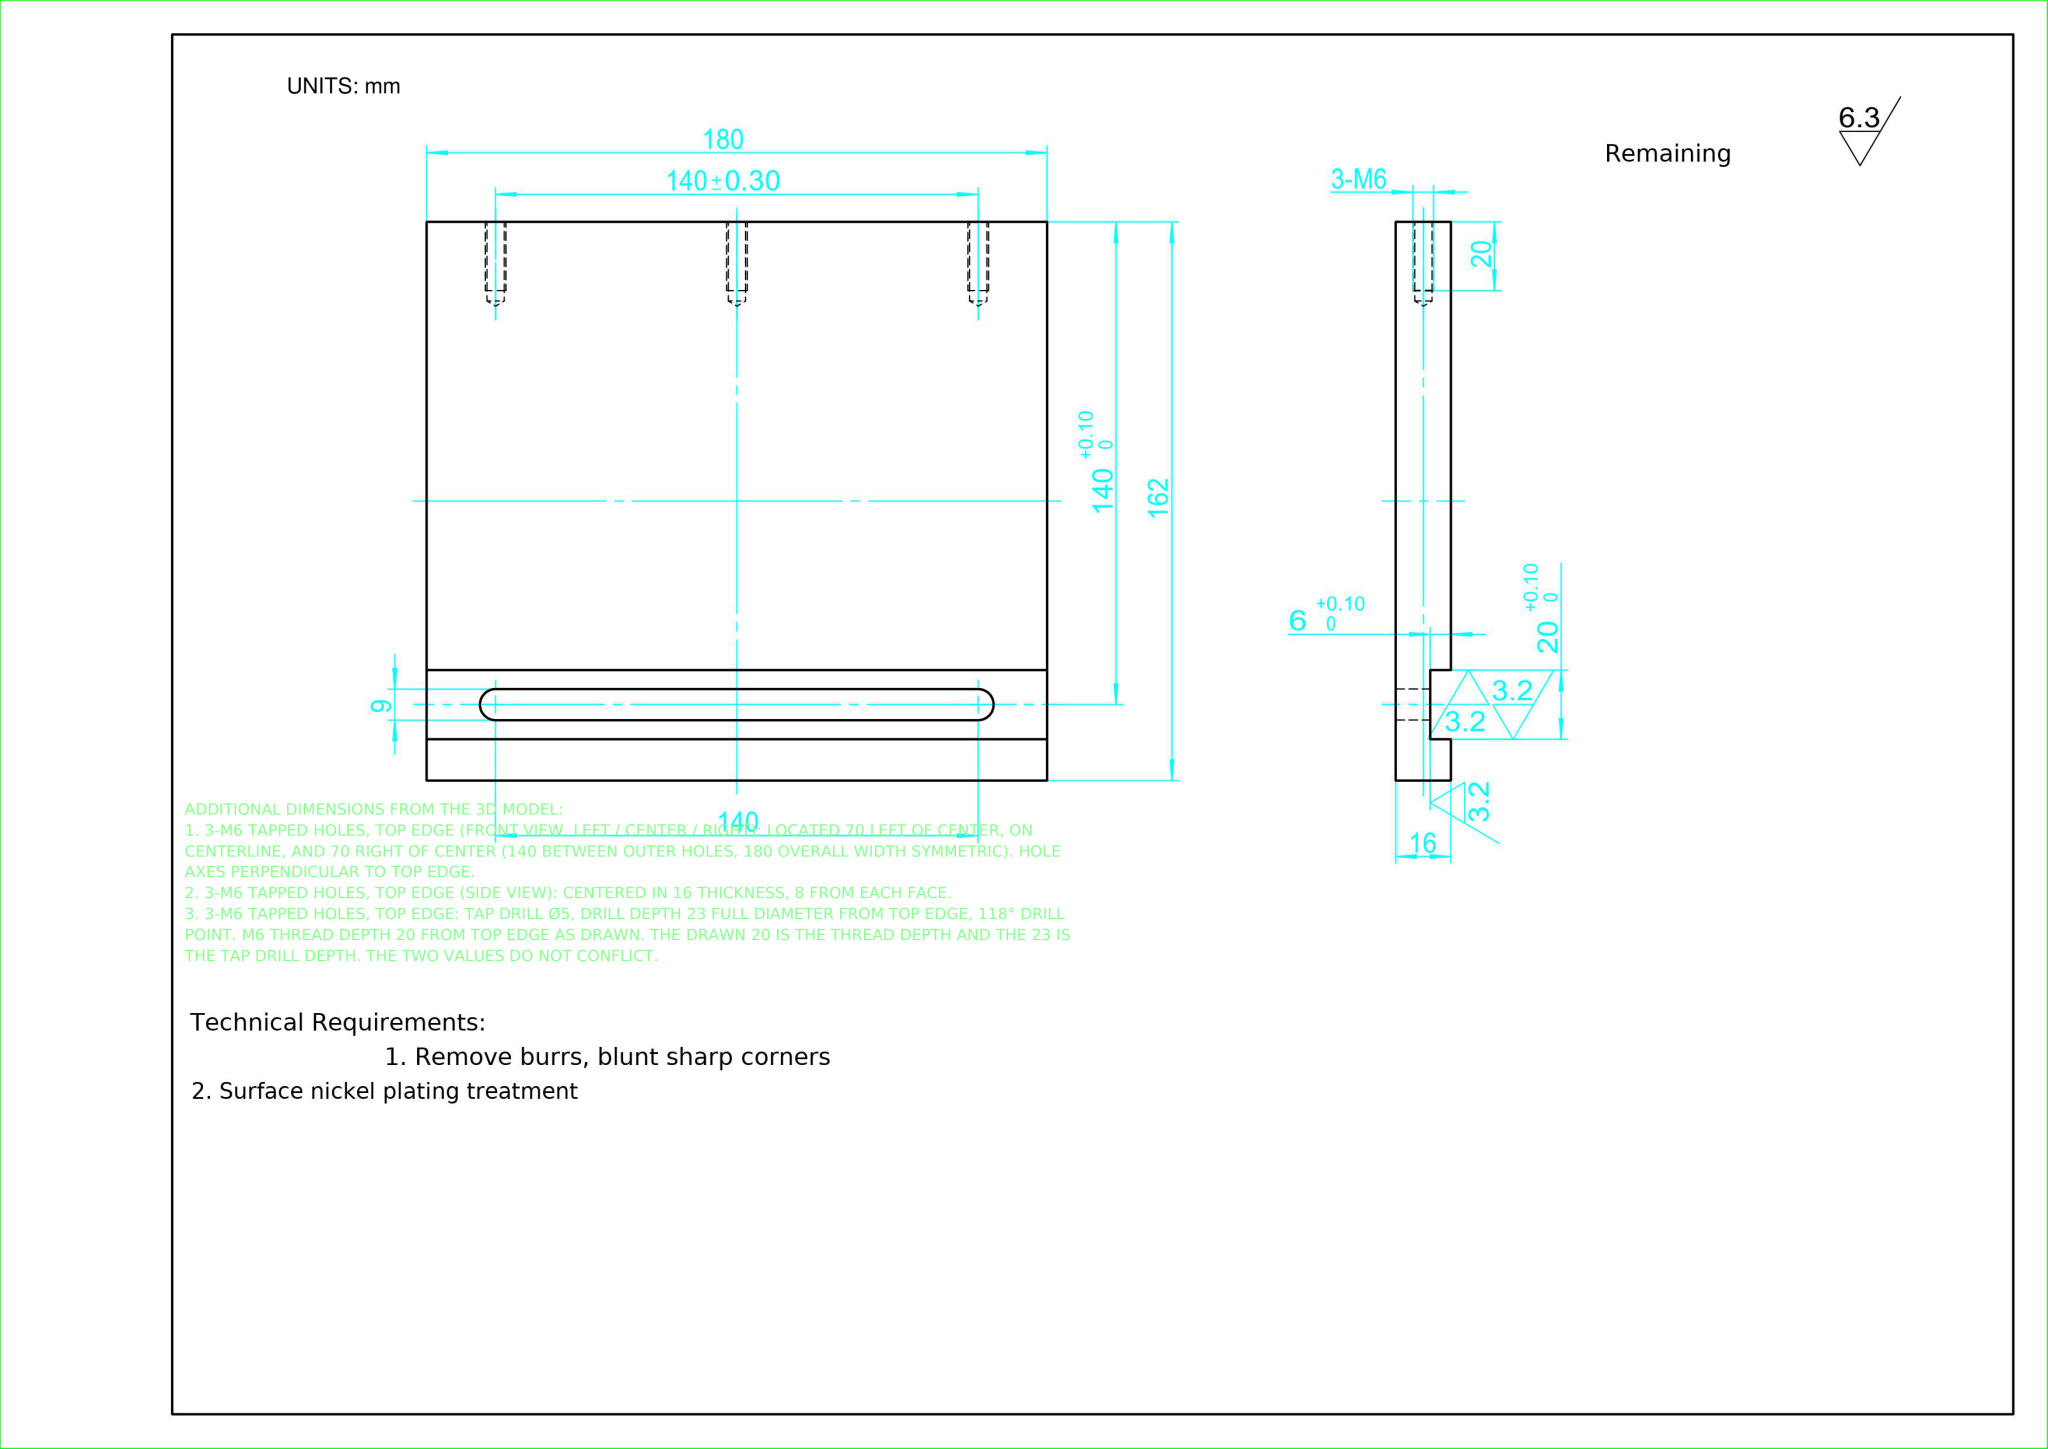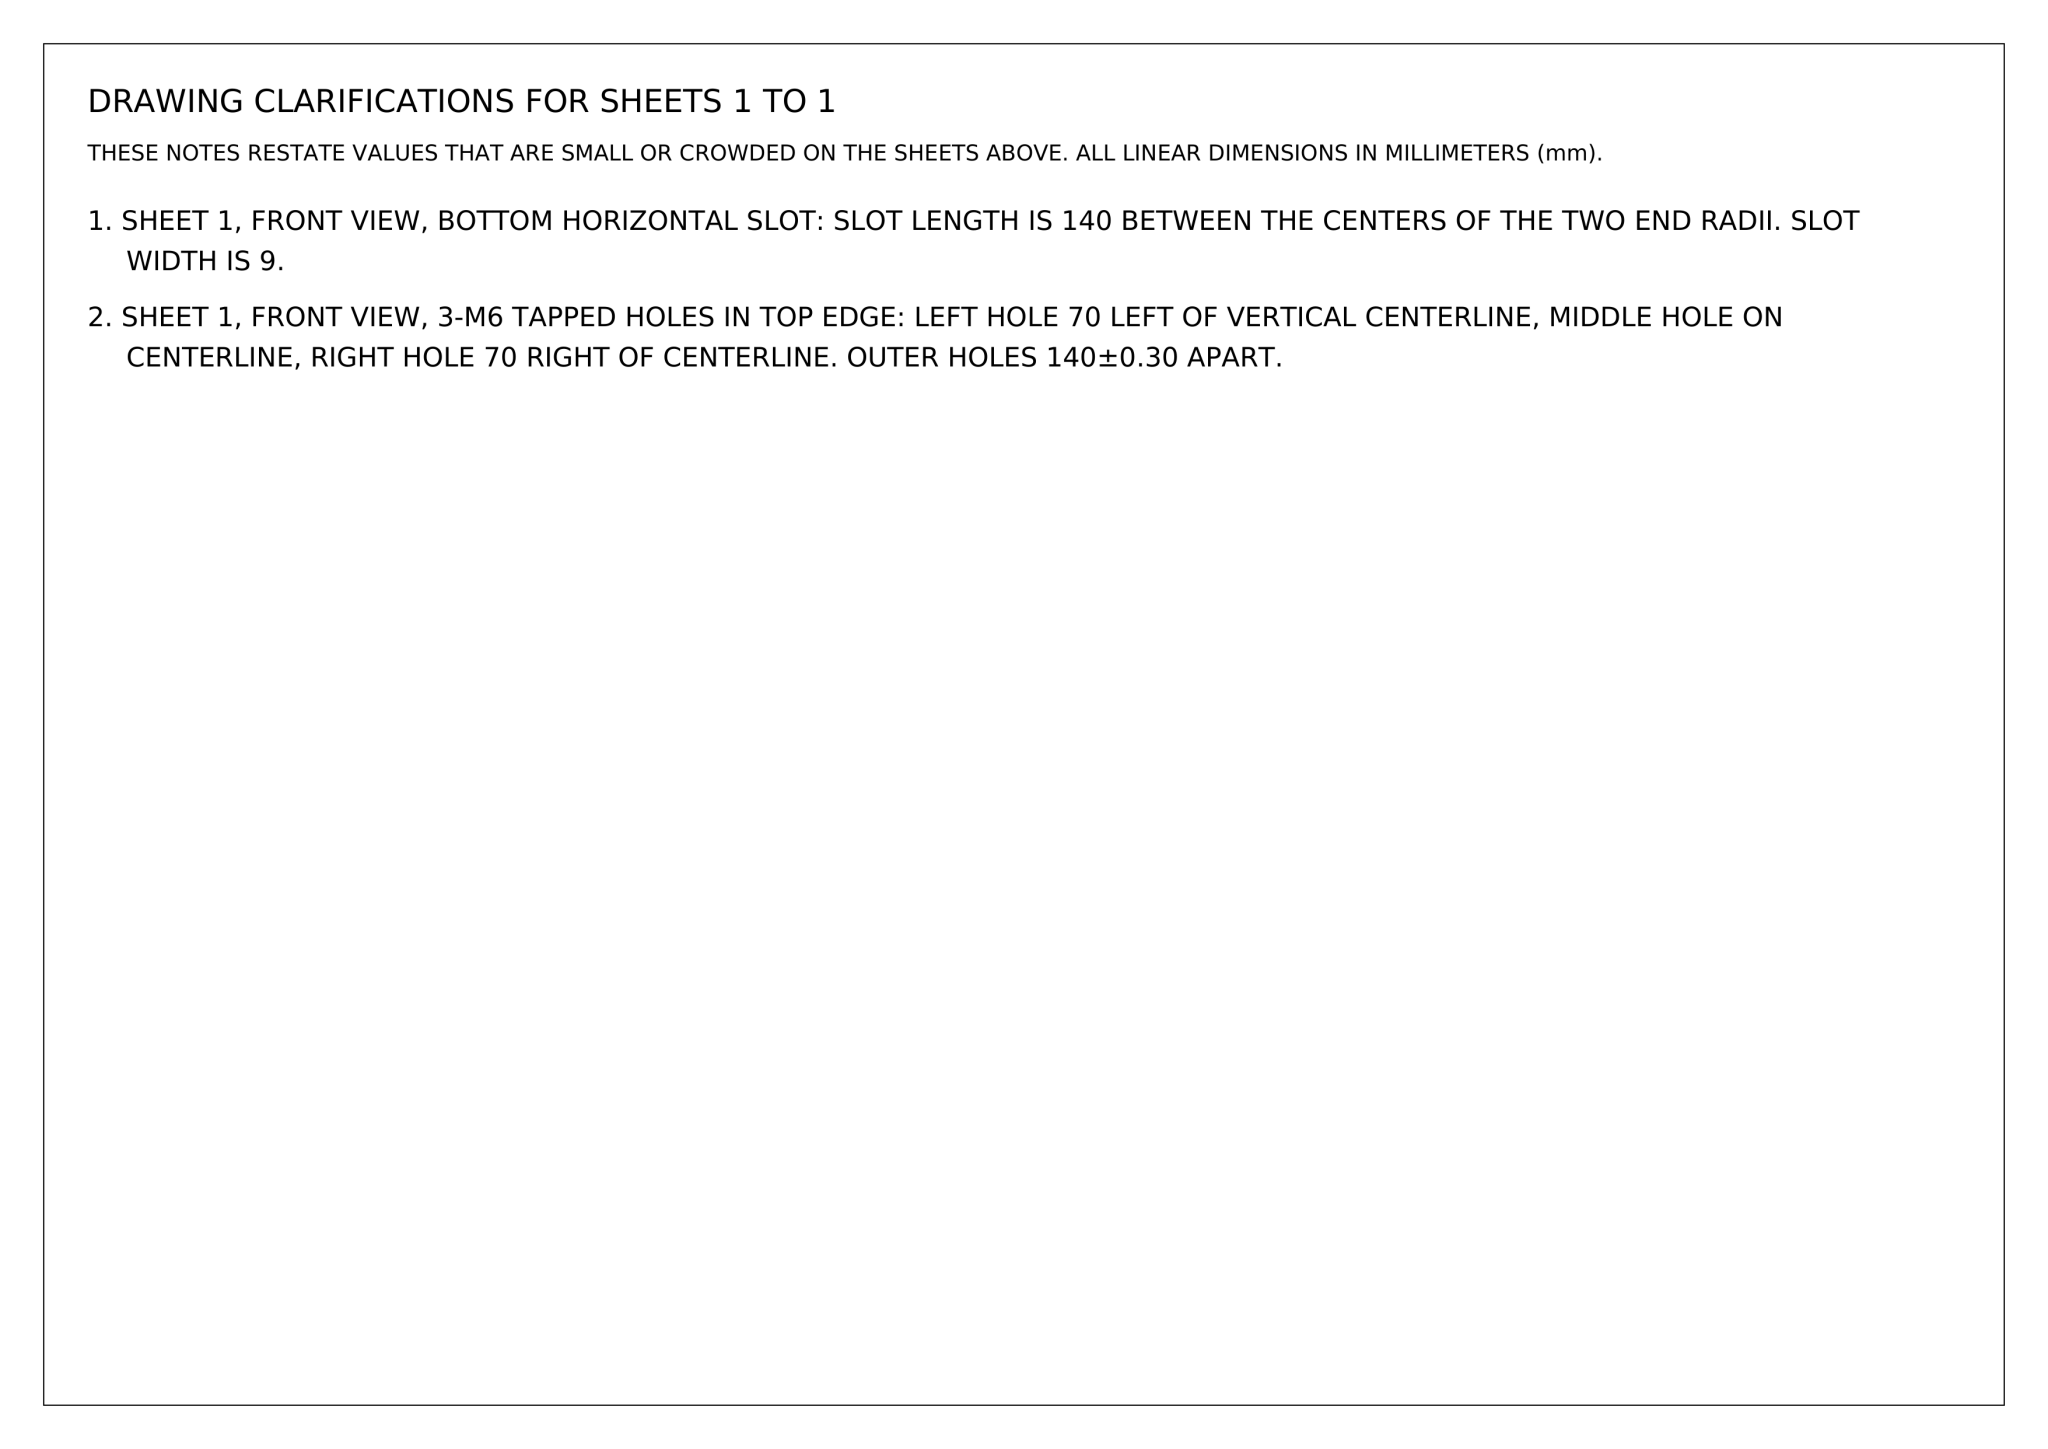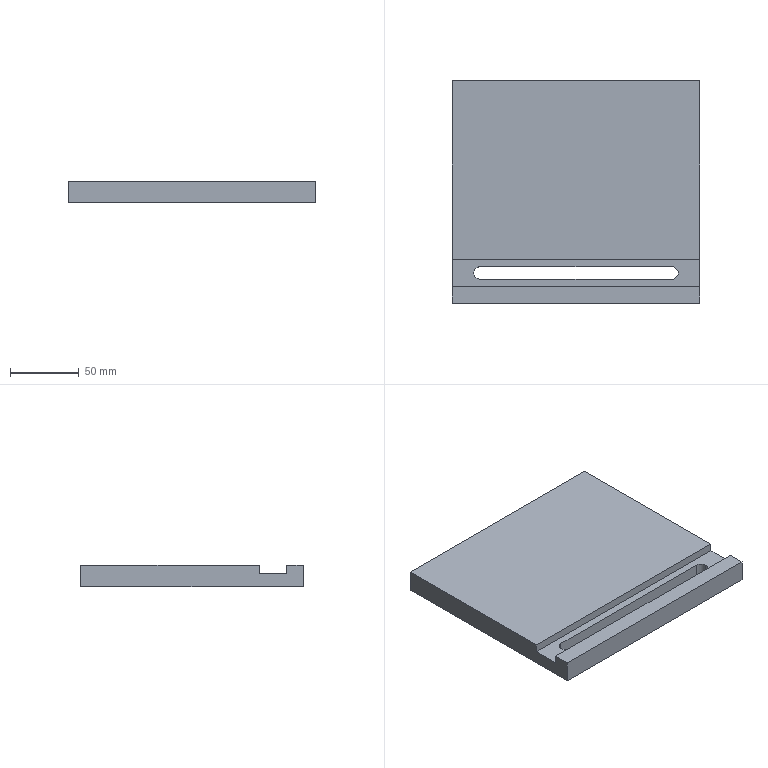Part | NX | mm | 1 solid | 27 faces | box 180 x 162 x 16 mm | volume 430340 mm3 | plane 12 | cylinder 9 | cone 6 | commonest cylinder face diameters 5 x6 9 x3